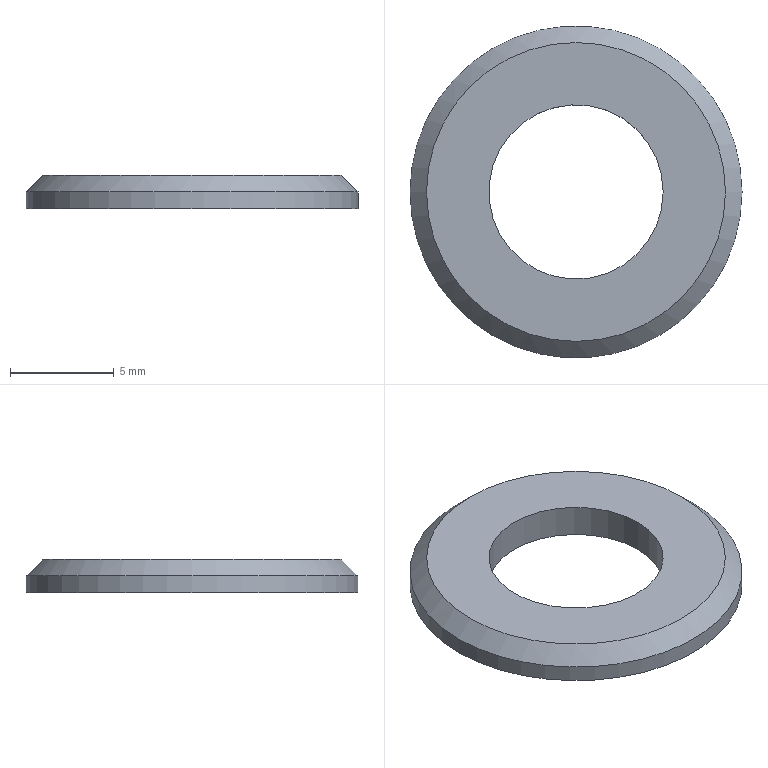Component | NX | GB-T97_2-2002_M8 | 1 solid | 5 faces | box 16 x 16 x 1.6 mm | volume 217 mm3 | cylinder 2 | plane 2 | cone 1 | commonest cylinder face diameters 16 x1 8.4 x1
STEP:
#1=CARTESIAN_POINT('',(0.,0.,0.));
#2=DIRECTION('',(0.,0.,1.));
#3=DIRECTION('',(1.,0.,0.));
#4=AXIS2_PLACEMENT_3D('',#1,#2,#3);
#5=CARTESIAN_POINT('',(-80.,45.,-185.2));
#6=VERTEX_POINT('',#5);
#7=CARTESIAN_POINT('',(-88.,45.,-185.2));
#8=DIRECTION('',(0.,0.,-1.));
#9=DIRECTION('',(1.,0.,0.));
#10=AXIS2_PLACEMENT_3D('',#7,#8,#9);
#11=CIRCLE('',#10,8.);
#12=CARTESIAN_POINT('',(-88.,45.,-184.4));
#13=DIRECTION('',(0.,0.,-1.));
#14=DIRECTION('',(-1.,0.,0.));
#15=AXIS2_PLACEMENT_3D('',#12,#13,#14);
#16=CYLINDRICAL_SURFACE('',#15,8.);
#17=CARTESIAN_POINT('',(3.142,0.8));
#18=DIRECTION('',(1.,0.));
#19=VECTOR('',#18,1.);
#20=LINE('',#17,#19);
#21=(GEOMETRIC_REPRESENTATION_CONTEXT(2)PARAMETRIC_REPRESENTATION_CONTEXT()REPRESENTATION_CONTEXT('',''));
#22=DEFINITIONAL_REPRESENTATION('',(#20),#21);
#23=PCURVE('',#16,#22);
#24=CARTESIAN_POINT('',(-88.,45.,-184.4));
#25=DIRECTION('',(0.,0.,-1.));
#26=DIRECTION('',(-1.,0.,0.));
#27=AXIS2_PLACEMENT_3D('',#24,#25,#26);
#28=CONICAL_SURFACE('',#27,7.2,0.7854);
#29=CARTESIAN_POINT('',(3.142,0.8));
#30=DIRECTION('',(1.,0.));
#31=VECTOR('',#30,1.);
#32=LINE('',#29,#31);
#33=(GEOMETRIC_REPRESENTATION_CONTEXT(2)PARAMETRIC_REPRESENTATION_CONTEXT()REPRESENTATION_CONTEXT('',''));
#34=DEFINITIONAL_REPRESENTATION('',(#32),#33);
#35=PCURVE('',#28,#34);
#36=SURFACE_CURVE('',#11,(#23,#35),.PCURVE_S1.);
#37=EDGE_CURVE('',#6,#6,#36,.T.);
#38=ORIENTED_EDGE('',*,*,#37,.T.);
#39=CARTESIAN_POINT('',(-80.,45.,-186.));
#40=VERTEX_POINT('',#39);
#41=CARTESIAN_POINT('',(-80.,45.,-185.2));
#42=CARTESIAN_POINT('',(-80.,45.,-186.));
#43=B_SPLINE_CURVE_WITH_KNOTS('',1,(#41,#42),.UNSPECIFIED.,.F.,.F.,(2,2),(0.8,1.6),.PIECEWISE_BEZIER_KNOTS.);
#44=CARTESIAN_POINT('',(9.425,0.));
#45=DIRECTION('',(0.,1.));
#46=VECTOR('',#45,1.);
#47=LINE('',#44,#46);
#48=(GEOMETRIC_REPRESENTATION_CONTEXT(2)PARAMETRIC_REPRESENTATION_CONTEXT()REPRESENTATION_CONTEXT('',''));
#49=DEFINITIONAL_REPRESENTATION('',(#47),#48);
#50=PCURVE('',#16,#49);
#51=CARTESIAN_POINT('',(3.142,0.));
#52=DIRECTION('',(0.,1.));
#53=VECTOR('',#52,1.);
#54=LINE('',#51,#53);
#55=(GEOMETRIC_REPRESENTATION_CONTEXT(2)PARAMETRIC_REPRESENTATION_CONTEXT()REPRESENTATION_CONTEXT('',''));
#56=DEFINITIONAL_REPRESENTATION('',(#54),#55);
#57=PCURVE('',#16,#56);
#58=SEAM_CURVE('',#43,(#50,#57),.PCURVE_S1.);
#59=EDGE_CURVE('',#6,#40,#58,.T.);
#60=ORIENTED_EDGE('',*,*,#59,.T.);
#61=CARTESIAN_POINT('',(-88.,45.,-186.));
#62=DIRECTION('',(0.,0.,1.));
#63=DIRECTION('',(1.,0.,0.));
#64=AXIS2_PLACEMENT_3D('',#61,#62,#63);
#65=CIRCLE('',#64,8.);
#66=CARTESIAN_POINT('',(9.425,1.6));
#67=DIRECTION('',(-1.,0.));
#68=VECTOR('',#67,1.);
#69=LINE('',#66,#68);
#70=(GEOMETRIC_REPRESENTATION_CONTEXT(2)PARAMETRIC_REPRESENTATION_CONTEXT()REPRESENTATION_CONTEXT('',''));
#71=DEFINITIONAL_REPRESENTATION('',(#69),#70);
#72=PCURVE('',#16,#71);
#73=CARTESIAN_POINT('',(-88.,45.,-186.));
#74=DIRECTION('',(0.,0.,1.));
#75=DIRECTION('',(1.,0.,0.));
#76=AXIS2_PLACEMENT_3D('',#73,#74,#75);
#77=PLANE('',#76);
#78=CARTESIAN_POINT('',(0.,0.));
#79=DIRECTION('',(1.,0.));
#80=AXIS2_PLACEMENT_2D('',#78,#79);
#81=CIRCLE('',#80,8.);
#82=(GEOMETRIC_REPRESENTATION_CONTEXT(2)PARAMETRIC_REPRESENTATION_CONTEXT()REPRESENTATION_CONTEXT('',''));
#83=DEFINITIONAL_REPRESENTATION('',(#81),#82);
#84=PCURVE('',#77,#83);
#85=SURFACE_CURVE('',#65,(#72,#84),.PCURVE_S1.);
#86=EDGE_CURVE('',#40,#40,#85,.T.);
#87=ORIENTED_EDGE('',*,*,#86,.T.);
#88=ORIENTED_EDGE('',*,*,#59,.F.);
#89=EDGE_LOOP('',(#38,#60,#87,#88));
#90=FACE_BOUND('',#89,.T.);
#91=ADVANCED_FACE('',(#90),#16,.T.);
#92=CARTESIAN_POINT('',(-83.8,45.,-184.4));
#93=VERTEX_POINT('',#92);
#94=CARTESIAN_POINT('',(-88.,45.,-184.4));
#95=DIRECTION('',(0.,0.,1.));
#96=DIRECTION('',(1.,0.,0.));
#97=AXIS2_PLACEMENT_3D('',#94,#95,#96);
#98=CIRCLE('',#97,4.2);
#99=CARTESIAN_POINT('',(-88.,45.,-184.4));
#100=DIRECTION('',(0.,0.,-1.));
#101=DIRECTION('',(-1.,0.,0.));
#102=AXIS2_PLACEMENT_3D('',#99,#100,#101);
#103=CYLINDRICAL_SURFACE('',#102,4.2);
#104=CARTESIAN_POINT('',(9.425,0.));
#105=DIRECTION('',(-1.,0.));
#106=VECTOR('',#105,1.);
#107=LINE('',#104,#106);
#108=(GEOMETRIC_REPRESENTATION_CONTEXT(2)PARAMETRIC_REPRESENTATION_CONTEXT()REPRESENTATION_CONTEXT('',''));
#109=DEFINITIONAL_REPRESENTATION('',(#107),#108);
#110=PCURVE('',#103,#109);
#111=CARTESIAN_POINT('',(-88.,45.,-184.4));
#112=DIRECTION('',(0.,0.,1.));
#113=DIRECTION('',(1.,0.,0.));
#114=AXIS2_PLACEMENT_3D('',#111,#112,#113);
#115=PLANE('',#114);
#116=CARTESIAN_POINT('',(0.,0.));
#117=DIRECTION('',(1.,0.));
#118=AXIS2_PLACEMENT_2D('',#116,#117);
#119=CIRCLE('',#118,4.2);
#120=(GEOMETRIC_REPRESENTATION_CONTEXT(2)PARAMETRIC_REPRESENTATION_CONTEXT()REPRESENTATION_CONTEXT('',''));
#121=DEFINITIONAL_REPRESENTATION('',(#119),#120);
#122=PCURVE('',#115,#121);
#123=SURFACE_CURVE('',#98,(#110,#122),.PCURVE_S1.);
#124=EDGE_CURVE('',#93,#93,#123,.T.);
#125=ORIENTED_EDGE('',*,*,#124,.F.);
#126=CARTESIAN_POINT('',(-83.8,45.,-186.));
#127=VERTEX_POINT('',#126);
#128=CARTESIAN_POINT('',(-83.8,45.,-184.4));
#129=CARTESIAN_POINT('',(-83.8,45.,-186.));
#130=B_SPLINE_CURVE_WITH_KNOTS('',1,(#128,#129),.UNSPECIFIED.,.F.,.F.,(2,2),(0.,1.6),.PIECEWISE_BEZIER_KNOTS.);
#131=CARTESIAN_POINT('',(9.425,0.));
#132=DIRECTION('',(0.,1.));
#133=VECTOR('',#132,1.);
#134=LINE('',#131,#133);
#135=(GEOMETRIC_REPRESENTATION_CONTEXT(2)PARAMETRIC_REPRESENTATION_CONTEXT()REPRESENTATION_CONTEXT('',''));
#136=DEFINITIONAL_REPRESENTATION('',(#134),#135);
#137=PCURVE('',#103,#136);
#138=CARTESIAN_POINT('',(3.142,0.));
#139=DIRECTION('',(0.,1.));
#140=VECTOR('',#139,1.);
#141=LINE('',#138,#140);
#142=(GEOMETRIC_REPRESENTATION_CONTEXT(2)PARAMETRIC_REPRESENTATION_CONTEXT()REPRESENTATION_CONTEXT('',''));
#143=DEFINITIONAL_REPRESENTATION('',(#141),#142);
#144=PCURVE('',#103,#143);
#145=SEAM_CURVE('',#130,(#137,#144),.PCURVE_S1.);
#146=EDGE_CURVE('',#93,#127,#145,.T.);
#147=ORIENTED_EDGE('',*,*,#146,.T.);
#148=CARTESIAN_POINT('',(-88.,45.,-186.));
#149=DIRECTION('',(0.,0.,1.));
#150=DIRECTION('',(1.,0.,0.));
#151=AXIS2_PLACEMENT_3D('',#148,#149,#150);
#152=CIRCLE('',#151,4.2);
#153=CARTESIAN_POINT('',(9.425,1.6));
#154=DIRECTION('',(-1.,0.));
#155=VECTOR('',#154,1.);
#156=LINE('',#153,#155);
#157=(GEOMETRIC_REPRESENTATION_CONTEXT(2)PARAMETRIC_REPRESENTATION_CONTEXT()REPRESENTATION_CONTEXT('',''));
#158=DEFINITIONAL_REPRESENTATION('',(#156),#157);
#159=PCURVE('',#103,#158);
#160=CARTESIAN_POINT('',(0.,0.));
#161=DIRECTION('',(1.,0.));
#162=AXIS2_PLACEMENT_2D('',#160,#161);
#163=CIRCLE('',#162,4.2);
#164=(GEOMETRIC_REPRESENTATION_CONTEXT(2)PARAMETRIC_REPRESENTATION_CONTEXT()REPRESENTATION_CONTEXT('',''));
#165=DEFINITIONAL_REPRESENTATION('',(#163),#164);
#166=PCURVE('',#77,#165);
#167=SURFACE_CURVE('',#152,(#159,#166),.PCURVE_S1.);
#168=EDGE_CURVE('',#127,#127,#167,.T.);
#169=ORIENTED_EDGE('',*,*,#168,.T.);
#170=ORIENTED_EDGE('',*,*,#146,.F.);
#171=EDGE_LOOP('',(#125,#147,#169,#170));
#172=FACE_BOUND('',#171,.F.);
#173=ADVANCED_FACE('',(#172),#103,.F.);
#174=CARTESIAN_POINT('',(-80.8,45.,-184.4));
#175=VERTEX_POINT('',#174);
#176=CARTESIAN_POINT('',(-88.,45.,-184.4));
#177=DIRECTION('',(0.,0.,1.));
#178=DIRECTION('',(1.,0.,0.));
#179=AXIS2_PLACEMENT_3D('',#176,#177,#178);
#180=CIRCLE('',#179,7.2);
#181=CARTESIAN_POINT('',(0.,0.));
#182=DIRECTION('',(1.,0.));
#183=AXIS2_PLACEMENT_2D('',#181,#182);
#184=CIRCLE('',#183,7.2);
#185=(GEOMETRIC_REPRESENTATION_CONTEXT(2)PARAMETRIC_REPRESENTATION_CONTEXT()REPRESENTATION_CONTEXT('',''));
#186=DEFINITIONAL_REPRESENTATION('',(#184),#185);
#187=PCURVE('',#115,#186);
#188=CARTESIAN_POINT('',(9.425,0.));
#189=DIRECTION('',(-1.,0.));
#190=VECTOR('',#189,1.);
#191=LINE('',#188,#190);
#192=(GEOMETRIC_REPRESENTATION_CONTEXT(2)PARAMETRIC_REPRESENTATION_CONTEXT()REPRESENTATION_CONTEXT('',''));
#193=DEFINITIONAL_REPRESENTATION('',(#191),#192);
#194=PCURVE('',#28,#193);
#195=SURFACE_CURVE('',#180,(#187,#194),.PCURVE_S1.);
#196=EDGE_CURVE('',#175,#175,#195,.T.);
#197=ORIENTED_EDGE('',*,*,#196,.T.);
#198=EDGE_LOOP('',(#197));
#199=FACE_BOUND('',#198,.T.);
#200=ORIENTED_EDGE('',*,*,#124,.F.);
#201=EDGE_LOOP('',(#200));
#202=FACE_BOUND('',#201,.T.);
#203=ADVANCED_FACE('',(#199,#202),#115,.T.);
#204=ORIENTED_EDGE('',*,*,#86,.F.);
#205=EDGE_LOOP('',(#204));
#206=FACE_BOUND('',#205,.T.);
#207=ORIENTED_EDGE('',*,*,#168,.T.);
#208=EDGE_LOOP('',(#207));
#209=FACE_BOUND('',#208,.T.);
#210=ADVANCED_FACE('',(#206,#209),#77,.F.);
#211=ORIENTED_EDGE('',*,*,#37,.F.);
#212=CARTESIAN_POINT('',(-80.8,45.,-184.4));
#213=CARTESIAN_POINT('',(-80.,45.,-185.2));
#214=B_SPLINE_CURVE_WITH_KNOTS('',1,(#212,#213),.UNSPECIFIED.,.F.,.F.,(2,2),(0.,1.131),.PIECEWISE_BEZIER_KNOTS.);
#215=CARTESIAN_POINT('',(3.142,0.));
#216=DIRECTION('',(0.,1.));
#217=VECTOR('',#216,1.);
#218=LINE('',#215,#217);
#219=(GEOMETRIC_REPRESENTATION_CONTEXT(2)PARAMETRIC_REPRESENTATION_CONTEXT()REPRESENTATION_CONTEXT('',''));
#220=DEFINITIONAL_REPRESENTATION('',(#218),#219);
#221=PCURVE('',#28,#220);
#222=CARTESIAN_POINT('',(9.425,0.));
#223=DIRECTION('',(0.,1.));
#224=VECTOR('',#223,1.);
#225=LINE('',#222,#224);
#226=(GEOMETRIC_REPRESENTATION_CONTEXT(2)PARAMETRIC_REPRESENTATION_CONTEXT()REPRESENTATION_CONTEXT('',''));
#227=DEFINITIONAL_REPRESENTATION('',(#225),#226);
#228=PCURVE('',#28,#227);
#229=SEAM_CURVE('',#214,(#221,#228),.PCURVE_S1.);
#230=EDGE_CURVE('',#175,#6,#229,.T.);
#231=ORIENTED_EDGE('',*,*,#230,.F.);
#232=ORIENTED_EDGE('',*,*,#196,.F.);
#233=ORIENTED_EDGE('',*,*,#230,.T.);
#234=EDGE_LOOP('',(#211,#231,#232,#233));
#235=FACE_BOUND('',#234,.T.);
#236=ADVANCED_FACE('',(#235),#28,.T.);
#237=CLOSED_SHELL('',(#91,#173,#203,#210,#236));
#238=MANIFOLD_SOLID_BREP('',#237);
#239=(LENGTH_UNIT()NAMED_UNIT(*)SI_UNIT(.MILLI.,.METRE.));
#240=UNCERTAINTY_MEASURE_WITH_UNIT(LENGTH_MEASURE(0.00001),#239,'','');
#241=(NAMED_UNIT(*)PLANE_ANGLE_UNIT()SI_UNIT($,.RADIAN.));
#242=(NAMED_UNIT(*)SI_UNIT($,.STERADIAN.)SOLID_ANGLE_UNIT());
#243=(GEOMETRIC_REPRESENTATION_CONTEXT(3)GLOBAL_UNCERTAINTY_ASSIGNED_CONTEXT((#240))GLOBAL_UNIT_ASSIGNED_CONTEXT((#239,#241,#242))REPRESENTATION_CONTEXT('',''));
#244=ADVANCED_BREP_SHAPE_REPRESENTATION('',(#4,#238),#243);